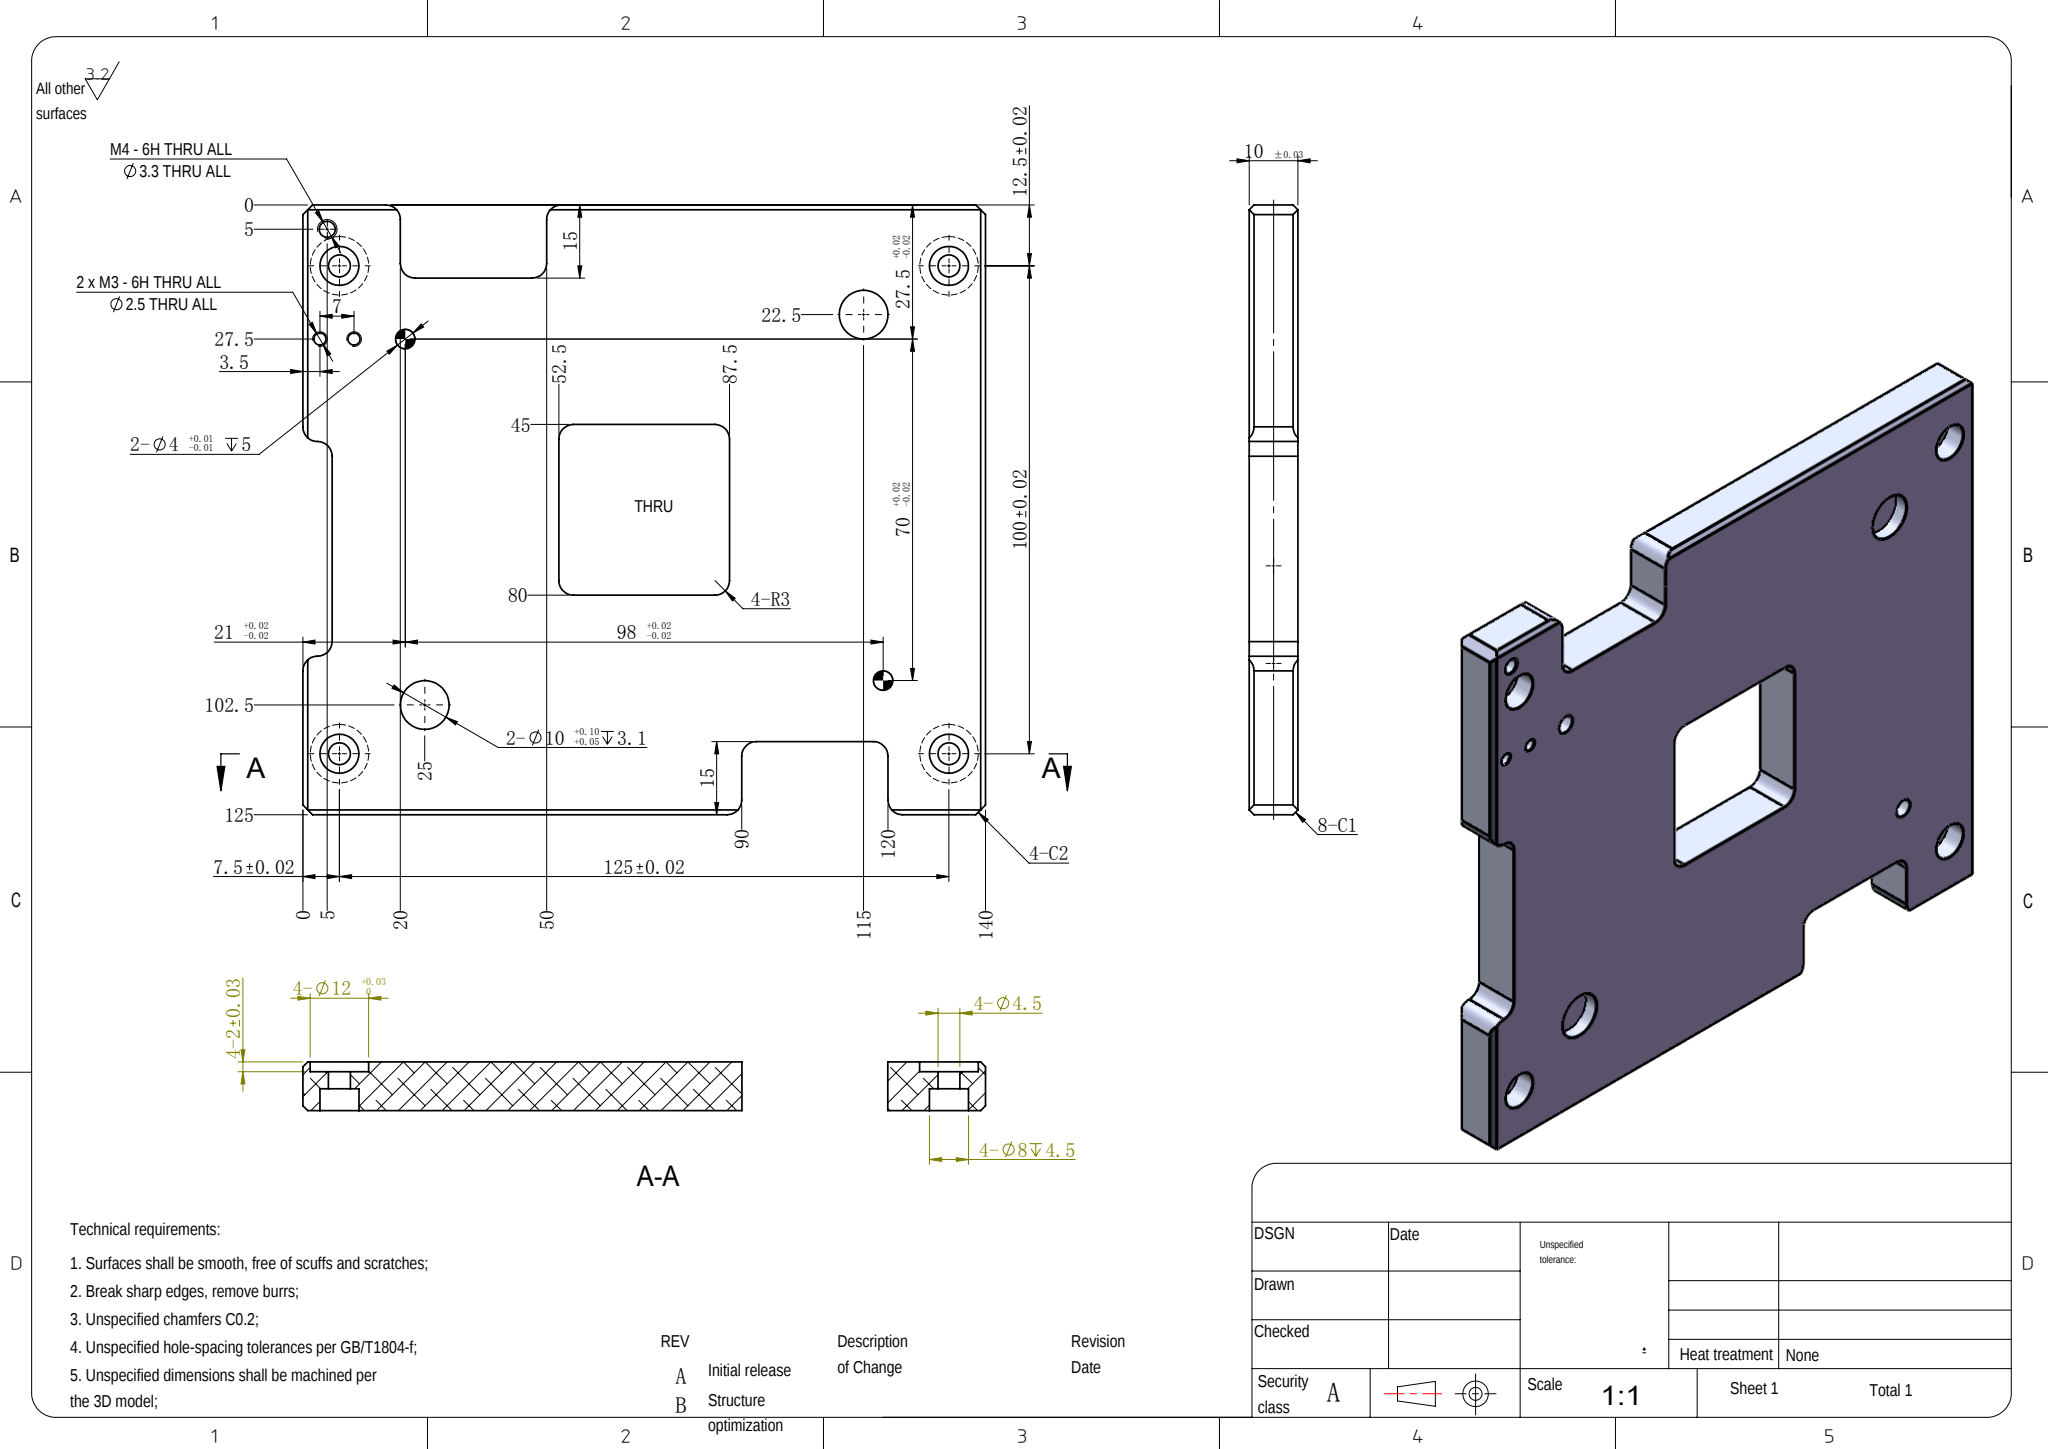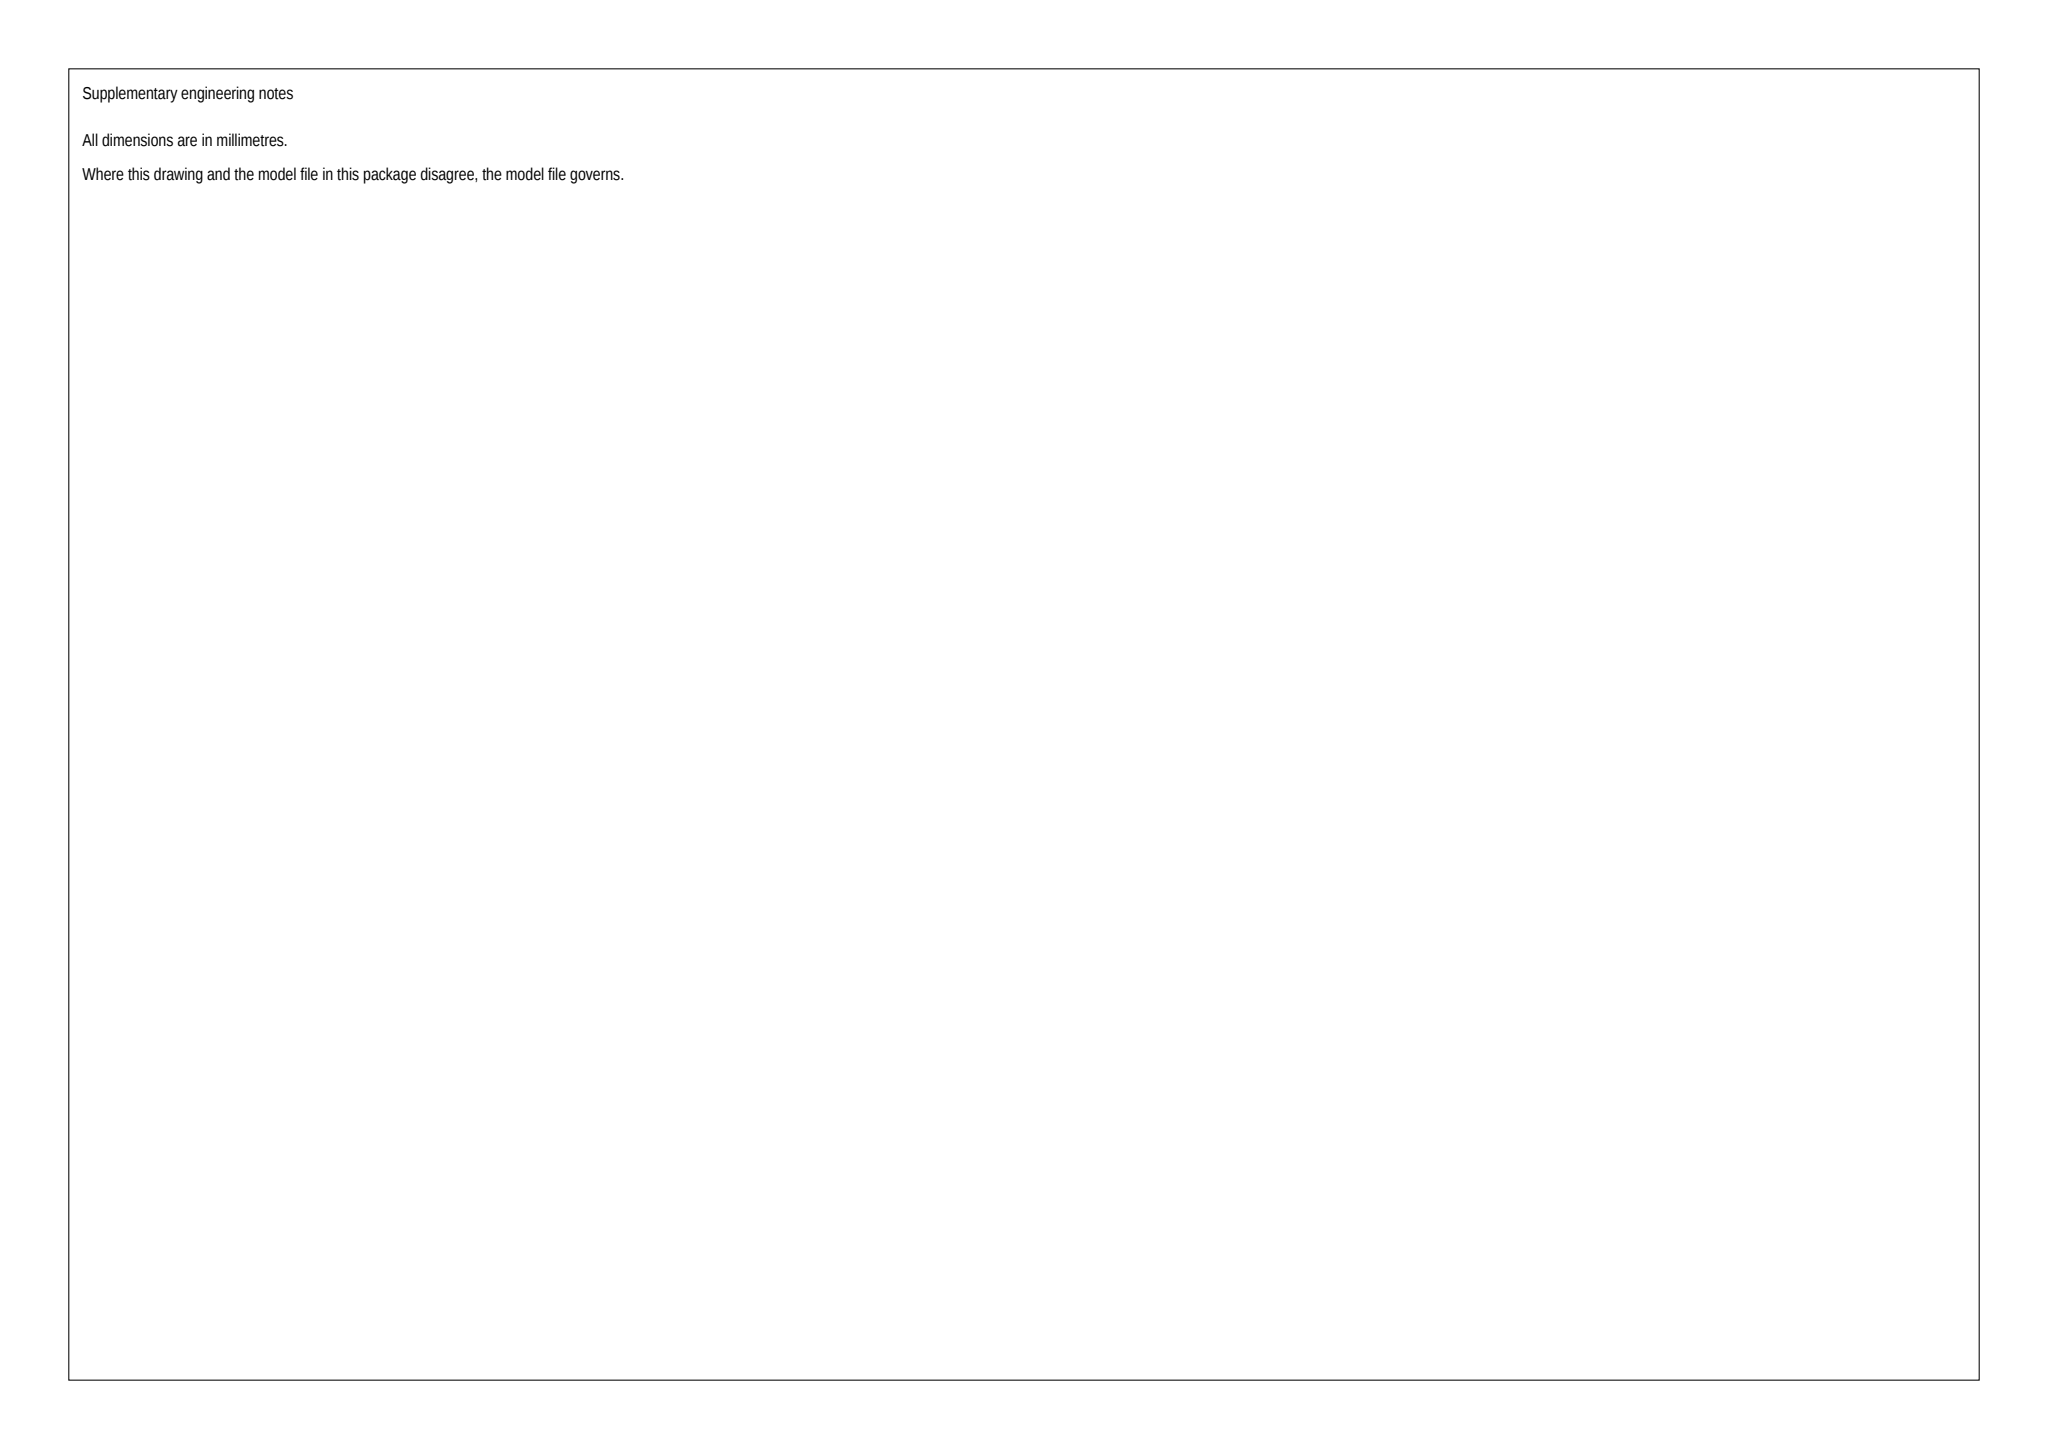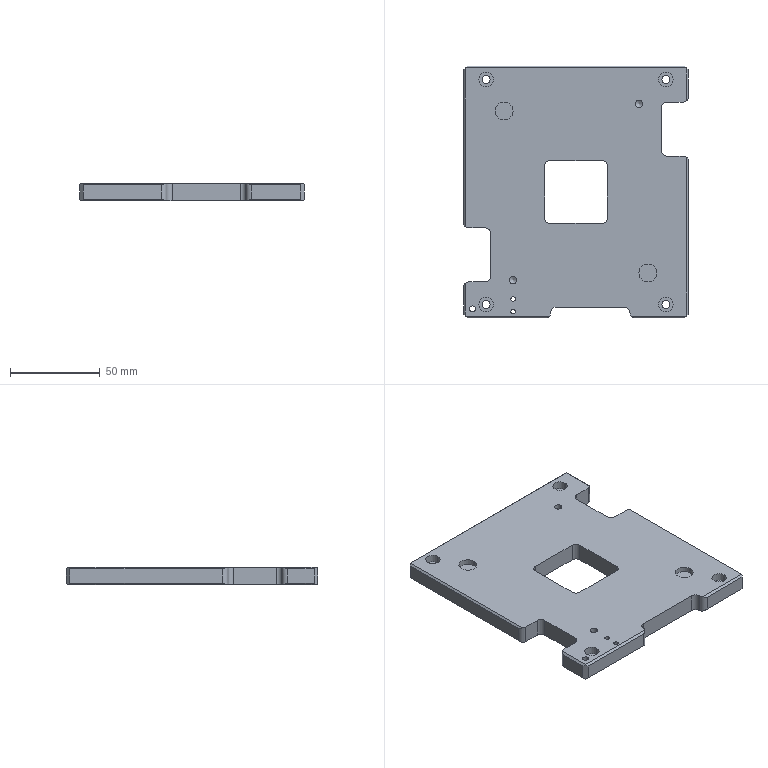Part | SolidWorks | mm | 1 solid | 106 faces | box 125 x 140 x 10 mm | volume 147866 mm3 | cylinder 54 | plane 48 | cone 4 | commonest cylinder face diameters 6 x16 12 x8 8 x8 4.5 x8 2.5 x4 10 x4 4 x4 3.3 x2